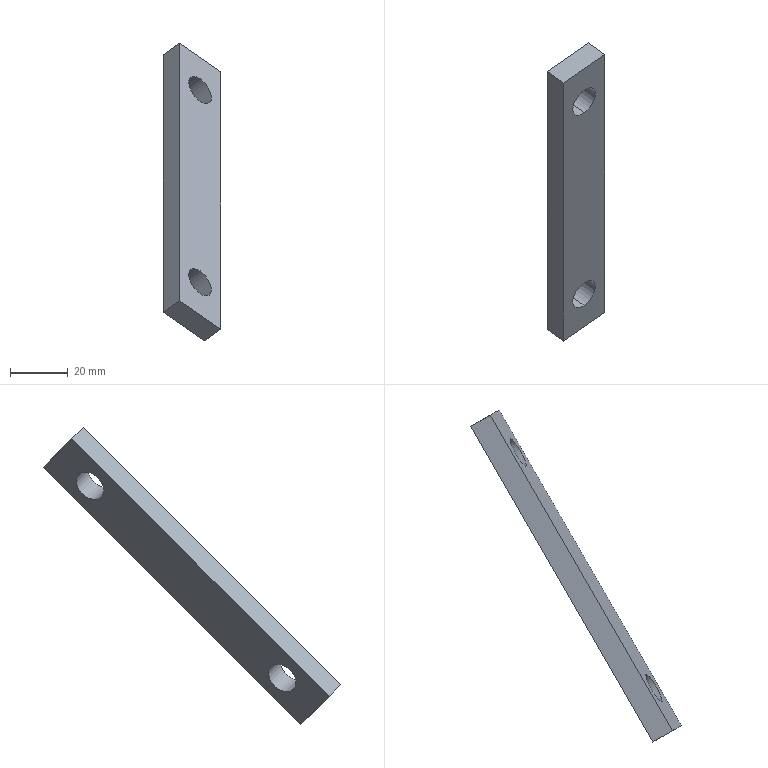Component | SolidWorks | SmallAxisAssembly-1_AdjustingRollerUpperPlate-1 | 1 solid | 10 faces | box 19.94 x 103.04 x 103.04 mm | volume 18639 mm3 | plane 6 | cylinder 4 | commonest cylinder face diameters 11 x4
build123d program:
from build123d import *

# Parameters (mm, degrees)
SKETCH1_W           = 126
SKETCH1_H           = 20
SKETCH1_R           = 5.5
BOSS_EXTRUDE1_DEPTH = 8


with BuildPart() as part:
    # Sketch1 → Boss-Extrude1 (new body)
    with BuildSketch(Plane.XY):
        Rectangle(SKETCH1_W, SKETCH1_H)
        with Locations((-47, 0)):
            Circle(SKETCH1_R, mode=Mode.SUBTRACT)
        with Locations((47, 0)):
            Circle(SKETCH1_R, mode=Mode.SUBTRACT)
    extrude(amount=BOSS_EXTRUDE1_DEPTH)


solid = part.part

# Placed as in the assembly
solid = solid.moved(Location((-22.138, 808.181, 240.989), (-134.971, -44.465, -89.958)))
STEP:
#1=COLOUR_RGB('',0.7922,0.8196,0.9333);
#2=FILL_AREA_STYLE_COLOUR('',#1);
#3=FILL_AREA_STYLE('',(#2));
#4=SURFACE_STYLE_FILL_AREA(#3);
#5=SURFACE_SIDE_STYLE('',(#4));
#6=SURFACE_STYLE_USAGE(.BOTH.,#5);
#7=PRESENTATION_STYLE_ASSIGNMENT((#6));
#8=CARTESIAN_POINT('',(-1.091,33.132,10.484));
#9=VERTEX_POINT('',#8);
#10=CARTESIAN_POINT('',(-1.091,33.439,10.79));
#11=VERTEX_POINT('',#10);
#12=CARTESIAN_POINT('',(-1.091,33.286,10.637));
#13=DIRECTION('',(-0.7005,0.5049,-0.5044));
#14=DIRECTION('',(0.0005225,0.7071,0.7071));
#15=AXIS2_PLACEMENT_3D('',#12,#13,#14);
#16=CIRCLE('',#15,0.2165);
#17=EDGE_CURVE('',#9,#11,#16,.T.);
#18=ORIENTED_EDGE('',*,*,#17,.T.);
#19=CARTESIAN_POINT('',(-0.8705,33.28,10.949));
#20=VERTEX_POINT('',#19);
#21=CARTESIAN_POINT('',(-1.091,33.439,10.79));
#22=DIRECTION('',(0.7005,-0.5049,0.5044));
#23=VECTOR('',#22,39.37);
#24=LINE('',#21,#23);
#25=EDGE_CURVE('',#11,#20,#24,.T.);
#26=ORIENTED_EDGE('',*,*,#25,.T.);
#27=CARTESIAN_POINT('',(-0.8707,32.973,10.643));
#28=VERTEX_POINT('',#27);
#29=CARTESIAN_POINT('',(-0.8706,33.127,10.796));
#30=DIRECTION('',(-0.7005,0.5049,-0.5044));
#31=DIRECTION('',(0.0005225,0.7071,0.7071));
#32=AXIS2_PLACEMENT_3D('',#29,#30,#31);
#33=CIRCLE('',#32,0.2165);
#34=EDGE_CURVE('',#28,#20,#33,.T.);
#35=ORIENTED_EDGE('',*,*,#34,.F.);
#36=CARTESIAN_POINT('',(-1.091,33.132,10.484));
#37=DIRECTION('',(0.7005,-0.5049,0.5044));
#38=VECTOR('',#37,39.37);
#39=LINE('',#36,#38);
#40=EDGE_CURVE('',#9,#28,#39,.T.);
#41=ORIENTED_EDGE('',*,*,#40,.F.);
#42=EDGE_LOOP('',(#18,#26,#35,#41));
#43=FACE_OUTER_BOUND('',#42,.T.);
#44=CARTESIAN_POINT('',(-1.091,33.286,10.637));
#45=DIRECTION('',(0.7005,-0.5049,0.5044));
#46=DIRECTION('',(-0.0005225,-0.7071,-0.7071));
#47=AXIS2_PLACEMENT_3D('',#44,#45,#46);
#48=CYLINDRICAL_SURFACE('',#47,0.2165);
#49=ADVANCED_FACE('',(#43),#48,.F.);
#50=CARTESIAN_POINT('',(-1.093,30.516,7.867));
#51=VERTEX_POINT('',#50);
#52=CARTESIAN_POINT('',(-1.093,30.822,8.174));
#53=VERTEX_POINT('',#52);
#54=CARTESIAN_POINT('',(-1.093,30.669,8.02));
#55=DIRECTION('',(-0.7005,0.5049,-0.5044));
#56=DIRECTION('',(0.0005225,0.7071,0.7071));
#57=AXIS2_PLACEMENT_3D('',#54,#55,#56);
#58=CIRCLE('',#57,0.2165);
#59=EDGE_CURVE('',#51,#53,#58,.T.);
#60=ORIENTED_EDGE('',*,*,#59,.T.);
#61=CARTESIAN_POINT('',(-0.8724,30.663,8.332));
#62=VERTEX_POINT('',#61);
#63=CARTESIAN_POINT('',(-1.093,30.822,8.174));
#64=DIRECTION('',(0.7005,-0.5049,0.5044));
#65=VECTOR('',#64,39.37);
#66=LINE('',#63,#65);
#67=EDGE_CURVE('',#53,#62,#66,.T.);
#68=ORIENTED_EDGE('',*,*,#67,.T.);
#69=CARTESIAN_POINT('',(-0.8727,30.357,8.026));
#70=VERTEX_POINT('',#69);
#71=CARTESIAN_POINT('',(-0.8725,30.51,8.179));
#72=DIRECTION('',(-0.7005,0.5049,-0.5044));
#73=DIRECTION('',(0.0005225,0.7071,0.7071));
#74=AXIS2_PLACEMENT_3D('',#71,#72,#73);
#75=CIRCLE('',#74,0.2165);
#76=EDGE_CURVE('',#70,#62,#75,.T.);
#77=ORIENTED_EDGE('',*,*,#76,.F.);
#78=CARTESIAN_POINT('',(-1.093,30.516,7.867));
#79=DIRECTION('',(0.7005,-0.5049,0.5044));
#80=VECTOR('',#79,39.37);
#81=LINE('',#78,#80);
#82=EDGE_CURVE('',#51,#70,#81,.T.);
#83=ORIENTED_EDGE('',*,*,#82,.F.);
#84=EDGE_LOOP('',(#60,#68,#77,#83));
#85=FACE_OUTER_BOUND('',#84,.T.);
#86=CARTESIAN_POINT('',(-1.093,30.669,8.02));
#87=DIRECTION('',(0.7005,-0.5049,0.5044));
#88=DIRECTION('',(-0.0005225,-0.7071,-0.7071));
#89=AXIS2_PLACEMENT_3D('',#86,#87,#88);
#90=CYLINDRICAL_SURFACE('',#89,0.2165);
#91=ADVANCED_FACE('',(#85),#90,.F.);
#92=CARTESIAN_POINT('',(-1.372,33.536,11.278));
#93=VERTEX_POINT('',#92);
#94=CARTESIAN_POINT('',(-0.8099,33.926,10.888));
#95=VERTEX_POINT('',#94);
#96=CARTESIAN_POINT('',(-1.372,33.536,11.278));
#97=DIRECTION('',(0.7137,0.495,-0.4956));
#98=VECTOR('',#97,39.37);
#99=LINE('',#96,#98);
#100=EDGE_CURVE('',#93,#95,#99,.T.);
#101=ORIENTED_EDGE('',*,*,#100,.T.);
#102=CARTESIAN_POINT('',(-0.8125,30.418,7.38));
#103=VERTEX_POINT('',#102);
#104=CARTESIAN_POINT('',(-0.8125,30.418,7.38));
#105=DIRECTION('',(-0.0005225,-0.7071,-0.7071));
#106=VECTOR('',#105,39.37);
#107=LINE('',#104,#106);
#108=EDGE_CURVE('',#95,#103,#107,.T.);
#109=ORIENTED_EDGE('',*,*,#108,.T.);
#110=CARTESIAN_POINT('',(-1.374,30.028,7.77));
#111=VERTEX_POINT('',#110);
#112=CARTESIAN_POINT('',(-1.374,30.028,7.77));
#113=DIRECTION('',(-0.7137,-0.495,0.4956));
#114=VECTOR('',#113,39.37);
#115=LINE('',#112,#114);
#116=EDGE_CURVE('',#103,#111,#115,.T.);
#117=ORIENTED_EDGE('',*,*,#116,.T.);
#118=CARTESIAN_POINT('',(-1.374,30.028,7.77));
#119=DIRECTION('',(0.0005225,0.7071,0.7071));
#120=VECTOR('',#119,39.37);
#121=LINE('',#118,#120);
#122=EDGE_CURVE('',#111,#93,#121,.T.);
#123=ORIENTED_EDGE('',*,*,#122,.T.);
#124=EDGE_LOOP('',(#101,#109,#117,#123));
#125=FACE_OUTER_BOUND('',#124,.T.);
#126=ORIENTED_EDGE('',*,*,#59,.F.);
#127=CARTESIAN_POINT('',(-1.093,30.669,8.02));
#128=DIRECTION('',(-0.7005,0.5049,-0.5044));
#129=DIRECTION('',(0.0005225,0.7071,0.7071));
#130=AXIS2_PLACEMENT_3D('',#127,#128,#129);
#131=CIRCLE('',#130,0.2165);
#132=EDGE_CURVE('',#53,#51,#131,.T.);
#133=ORIENTED_EDGE('',*,*,#132,.F.);
#134=EDGE_LOOP('',(#126,#133));
#135=FACE_BOUND('',#134,.T.);
#136=ORIENTED_EDGE('',*,*,#17,.F.);
#137=CARTESIAN_POINT('',(-1.091,33.286,10.637));
#138=DIRECTION('',(-0.7005,0.5049,-0.5044));
#139=DIRECTION('',(0.0005225,0.7071,0.7071));
#140=AXIS2_PLACEMENT_3D('',#137,#138,#139);
#141=CIRCLE('',#140,0.2165);
#142=EDGE_CURVE('',#11,#9,#141,.T.);
#143=ORIENTED_EDGE('',*,*,#142,.F.);
#144=EDGE_LOOP('',(#136,#143));
#145=FACE_BOUND('',#144,.T.);
#146=CARTESIAN_POINT('',(-1.092,31.977,9.329));
#147=DIRECTION('',(0.7005,-0.5049,0.5044));
#148=DIRECTION('',(-0.0005225,-0.7071,-0.7071));
#149=AXIS2_PLACEMENT_3D('',#146,#147,#148);
#150=PLANE('',#149);
#151=ADVANCED_FACE('',(#125,#135,#145),#150,.F.);
#152=ORIENTED_EDGE('',*,*,#76,.T.);
#153=CARTESIAN_POINT('',(-0.8725,30.51,8.179));
#154=DIRECTION('',(-0.7005,0.5049,-0.5044));
#155=DIRECTION('',(0.0005225,0.7071,0.7071));
#156=AXIS2_PLACEMENT_3D('',#153,#154,#155);
#157=CIRCLE('',#156,0.2165);
#158=EDGE_CURVE('',#62,#70,#157,.T.);
#159=ORIENTED_EDGE('',*,*,#158,.T.);
#160=EDGE_LOOP('',(#152,#159));
#161=FACE_BOUND('',#160,.T.);
#162=CARTESIAN_POINT('',(-1.151,33.377,11.437));
#163=VERTEX_POINT('',#162);
#164=CARTESIAN_POINT('',(-0.5893,33.767,11.046));
#165=VERTEX_POINT('',#164);
#166=CARTESIAN_POINT('',(-1.151,33.377,11.437));
#167=DIRECTION('',(0.7137,0.495,-0.4956));
#168=VECTOR('',#167,39.37);
#169=LINE('',#166,#168);
#170=EDGE_CURVE('',#163,#165,#169,.T.);
#171=ORIENTED_EDGE('',*,*,#170,.F.);
#172=CARTESIAN_POINT('',(-1.154,29.869,7.929));
#173=VERTEX_POINT('',#172);
#174=CARTESIAN_POINT('',(-1.154,29.869,7.929));
#175=DIRECTION('',(0.0005225,0.7071,0.7071));
#176=VECTOR('',#175,39.37);
#177=LINE('',#174,#176);
#178=EDGE_CURVE('',#173,#163,#177,.T.);
#179=ORIENTED_EDGE('',*,*,#178,.F.);
#180=CARTESIAN_POINT('',(-0.5919,30.259,7.539));
#181=VERTEX_POINT('',#180);
#182=CARTESIAN_POINT('',(-1.154,29.869,7.929));
#183=DIRECTION('',(-0.7137,-0.495,0.4956));
#184=VECTOR('',#183,39.37);
#185=LINE('',#182,#184);
#186=EDGE_CURVE('',#181,#173,#185,.T.);
#187=ORIENTED_EDGE('',*,*,#186,.F.);
#188=CARTESIAN_POINT('',(-0.5919,30.259,7.539));
#189=DIRECTION('',(-0.0005225,-0.7071,-0.7071));
#190=VECTOR('',#189,39.37);
#191=LINE('',#188,#190);
#192=EDGE_CURVE('',#165,#181,#191,.T.);
#193=ORIENTED_EDGE('',*,*,#192,.F.);
#194=EDGE_LOOP('',(#171,#179,#187,#193));
#195=FACE_OUTER_BOUND('',#194,.T.);
#196=ORIENTED_EDGE('',*,*,#34,.T.);
#197=CARTESIAN_POINT('',(-0.8706,33.127,10.796));
#198=DIRECTION('',(-0.7005,0.5049,-0.5044));
#199=DIRECTION('',(0.0005225,0.7071,0.7071));
#200=AXIS2_PLACEMENT_3D('',#197,#198,#199);
#201=CIRCLE('',#200,0.2165);
#202=EDGE_CURVE('',#20,#28,#201,.T.);
#203=ORIENTED_EDGE('',*,*,#202,.T.);
#204=EDGE_LOOP('',(#196,#203));
#205=FACE_BOUND('',#204,.T.);
#206=CARTESIAN_POINT('',(-0.8716,31.818,9.488));
#207=DIRECTION('',(0.7005,-0.5049,0.5044));
#208=DIRECTION('',(-0.0005225,-0.7071,-0.7071));
#209=AXIS2_PLACEMENT_3D('',#206,#207,#208);
#210=PLANE('',#209);
#211=ADVANCED_FACE('',(#161,#195,#205),#210,.T.);
#212=ORIENTED_EDGE('',*,*,#170,.T.);
#213=CARTESIAN_POINT('',(-0.8099,33.926,10.888));
#214=DIRECTION('',(0.7005,-0.5049,0.5044));
#215=VECTOR('',#214,39.37);
#216=LINE('',#213,#215);
#217=EDGE_CURVE('',#95,#165,#216,.T.);
#218=ORIENTED_EDGE('',*,*,#217,.F.);
#219=ORIENTED_EDGE('',*,*,#100,.F.);
#220=CARTESIAN_POINT('',(-1.372,33.536,11.278));
#221=DIRECTION('',(0.7005,-0.5049,0.5044));
#222=VECTOR('',#221,39.37);
#223=LINE('',#220,#222);
#224=EDGE_CURVE('',#93,#163,#223,.T.);
#225=ORIENTED_EDGE('',*,*,#224,.T.);
#226=EDGE_LOOP('',(#212,#218,#219,#225));
#227=FACE_OUTER_BOUND('',#226,.T.);
#228=CARTESIAN_POINT('',(-1.372,33.536,11.278));
#229=DIRECTION('',(-0.0005225,-0.7071,-0.7071));
#230=DIRECTION('',(-0.7005,0.5049,-0.5044));
#231=AXIS2_PLACEMENT_3D('',#228,#229,#230);
#232=PLANE('',#231);
#233=ADVANCED_FACE('',(#227),#232,.F.);
#234=ORIENTED_EDGE('',*,*,#192,.T.);
#235=CARTESIAN_POINT('',(-0.8125,30.418,7.38));
#236=DIRECTION('',(0.7005,-0.5049,0.5044));
#237=VECTOR('',#236,39.37);
#238=LINE('',#235,#237);
#239=EDGE_CURVE('',#103,#181,#238,.T.);
#240=ORIENTED_EDGE('',*,*,#239,.F.);
#241=ORIENTED_EDGE('',*,*,#108,.F.);
#242=ORIENTED_EDGE('',*,*,#217,.T.);
#243=EDGE_LOOP('',(#234,#240,#241,#242));
#244=FACE_OUTER_BOUND('',#243,.T.);
#245=CARTESIAN_POINT('',(-0.8125,30.418,7.38));
#246=DIRECTION('',(-0.7137,-0.495,0.4956));
#247=DIRECTION('',(0.0005225,0.7071,0.7071));
#248=AXIS2_PLACEMENT_3D('',#245,#246,#247);
#249=PLANE('',#248);
#250=ADVANCED_FACE('',(#244),#249,.F.);
#251=ORIENTED_EDGE('',*,*,#186,.T.);
#252=CARTESIAN_POINT('',(-1.374,30.028,7.77));
#253=DIRECTION('',(0.7005,-0.5049,0.5044));
#254=VECTOR('',#253,39.37);
#255=LINE('',#252,#254);
#256=EDGE_CURVE('',#111,#173,#255,.T.);
#257=ORIENTED_EDGE('',*,*,#256,.F.);
#258=ORIENTED_EDGE('',*,*,#116,.F.);
#259=ORIENTED_EDGE('',*,*,#239,.T.);
#260=EDGE_LOOP('',(#251,#257,#258,#259));
#261=FACE_OUTER_BOUND('',#260,.T.);
#262=CARTESIAN_POINT('',(-1.374,30.028,7.77));
#263=DIRECTION('',(0.0005225,0.7071,0.7071));
#264=DIRECTION('',(0.7005,-0.5049,0.5044));
#265=AXIS2_PLACEMENT_3D('',#262,#263,#264);
#266=PLANE('',#265);
#267=ADVANCED_FACE('',(#261),#266,.F.);
#268=ORIENTED_EDGE('',*,*,#178,.T.);
#269=ORIENTED_EDGE('',*,*,#224,.F.);
#270=ORIENTED_EDGE('',*,*,#122,.F.);
#271=ORIENTED_EDGE('',*,*,#256,.T.);
#272=EDGE_LOOP('',(#268,#269,#270,#271));
#273=FACE_OUTER_BOUND('',#272,.T.);
#274=CARTESIAN_POINT('',(-1.374,30.028,7.77));
#275=DIRECTION('',(0.7137,0.495,-0.4956));
#276=DIRECTION('',(-0.7005,0.5049,-0.5044));
#277=AXIS2_PLACEMENT_3D('',#274,#275,#276);
#278=PLANE('',#277);
#279=ADVANCED_FACE('',(#273),#278,.F.);
#280=ORIENTED_EDGE('',*,*,#67,.F.);
#281=ORIENTED_EDGE('',*,*,#132,.T.);
#282=ORIENTED_EDGE('',*,*,#82,.T.);
#283=ORIENTED_EDGE('',*,*,#158,.F.);
#284=EDGE_LOOP('',(#280,#281,#282,#283));
#285=FACE_OUTER_BOUND('',#284,.T.);
#286=CARTESIAN_POINT('',(-1.093,30.669,8.02));
#287=DIRECTION('',(0.7005,-0.5049,0.5044));
#288=DIRECTION('',(-0.0005225,-0.7071,-0.7071));
#289=AXIS2_PLACEMENT_3D('',#286,#287,#288);
#290=CYLINDRICAL_SURFACE('',#289,0.2165);
#291=ADVANCED_FACE('',(#285),#290,.F.);
#292=ORIENTED_EDGE('',*,*,#25,.F.);
#293=ORIENTED_EDGE('',*,*,#142,.T.);
#294=ORIENTED_EDGE('',*,*,#40,.T.);
#295=ORIENTED_EDGE('',*,*,#202,.F.);
#296=EDGE_LOOP('',(#292,#293,#294,#295));
#297=FACE_OUTER_BOUND('',#296,.T.);
#298=CARTESIAN_POINT('',(-1.091,33.286,10.637));
#299=DIRECTION('',(0.7005,-0.5049,0.5044));
#300=DIRECTION('',(-0.0005225,-0.7071,-0.7071));
#301=AXIS2_PLACEMENT_3D('',#298,#299,#300);
#302=CYLINDRICAL_SURFACE('',#301,0.2165);
#303=ADVANCED_FACE('',(#297),#302,.F.);
#304=CLOSED_SHELL('',(#49,#91,#151,#211,#233,#250,#267,#279,#291,#303));
#305=MANIFOLD_SOLID_BREP('',#304);
#306=STYLED_ITEM('',(#7),#305);
#307=PRESENTATION_LAYER_ASSIGNMENT('','',(#306));
#308=CARTESIAN_POINT('',(0.,0.,0.));
#309=DIRECTION('',(0.,0.,1.));
#310=DIRECTION('',(1.,0.,0.));
#311=AXIS2_PLACEMENT_3D('',#308,#309,#310);
#312=(LENGTH_UNIT()NAMED_UNIT(*)SI_UNIT($,.METRE.));
#313=LENGTH_MEASURE_WITH_UNIT(LENGTH_MEASURE(0.0254),#312);
#314=DIMENSIONAL_EXPONENTS(1.,0.,0.,0.,0.,0.,0.);
#315=(CONVERSION_BASED_UNIT('',#313)LENGTH_UNIT()NAMED_UNIT(#314));
#316=UNCERTAINTY_MEASURE_WITH_UNIT(LENGTH_MEASURE(0.00001),#315,'','');
#317=(NAMED_UNIT(*)PLANE_ANGLE_UNIT()SI_UNIT($,.RADIAN.));
#318=(NAMED_UNIT(*)SI_UNIT($,.STERADIAN.)SOLID_ANGLE_UNIT());
#319=(GEOMETRIC_REPRESENTATION_CONTEXT(3)GLOBAL_UNCERTAINTY_ASSIGNED_CONTEXT((#316))GLOBAL_UNIT_ASSIGNED_CONTEXT((#315,#317,#318))REPRESENTATION_CONTEXT('',''));
#320=ADVANCED_BREP_SHAPE_REPRESENTATION('',(#305,#311),#319);
#321=(LENGTH_UNIT()NAMED_UNIT(*)SI_UNIT($,.METRE.));
#322=LENGTH_MEASURE_WITH_UNIT(LENGTH_MEASURE(0.0254),#321);
#323=DIMENSIONAL_EXPONENTS(1.,0.,0.,0.,0.,0.,0.);
#324=(CONVERSION_BASED_UNIT('',#322)LENGTH_UNIT()NAMED_UNIT(#323));
#325=UNCERTAINTY_MEASURE_WITH_UNIT(LENGTH_MEASURE(0.00001),#324,'','');
#326=(NAMED_UNIT(*)PLANE_ANGLE_UNIT()SI_UNIT($,.RADIAN.));
#327=(NAMED_UNIT(*)SI_UNIT($,.STERADIAN.)SOLID_ANGLE_UNIT());
#328=(GEOMETRIC_REPRESENTATION_CONTEXT(3)GLOBAL_UNCERTAINTY_ASSIGNED_CONTEXT((#325))GLOBAL_UNIT_ASSIGNED_CONTEXT((#324,#326,#327))REPRESENTATION_CONTEXT('',''));
#329=MECHANICAL_DESIGN_GEOMETRIC_PRESENTATION_REPRESENTATION('',(#306),#328);